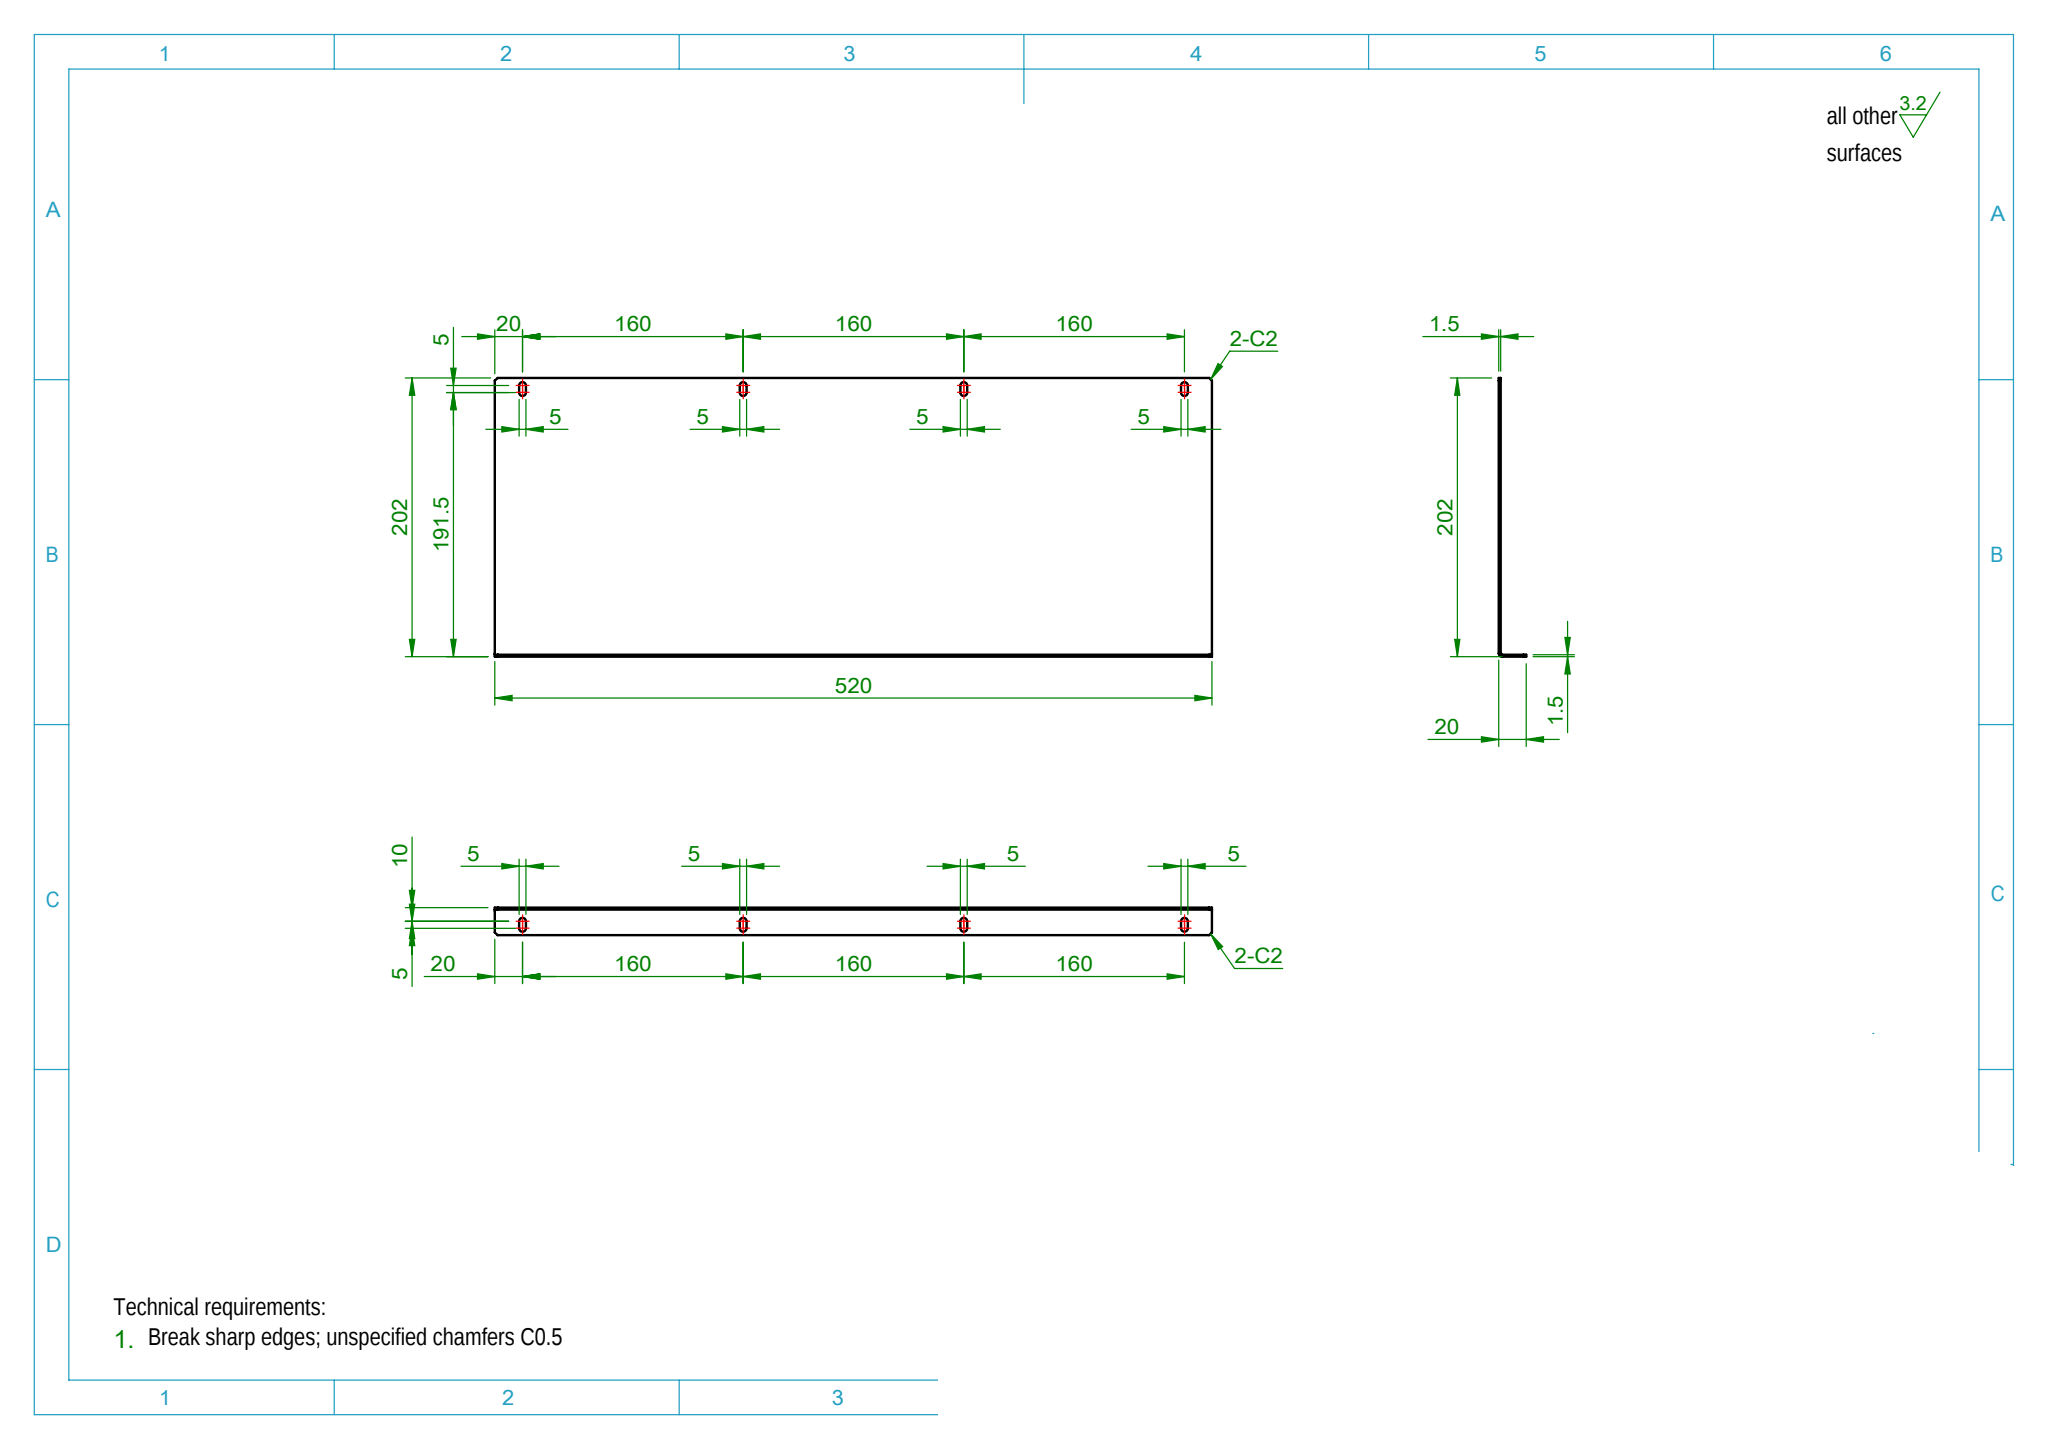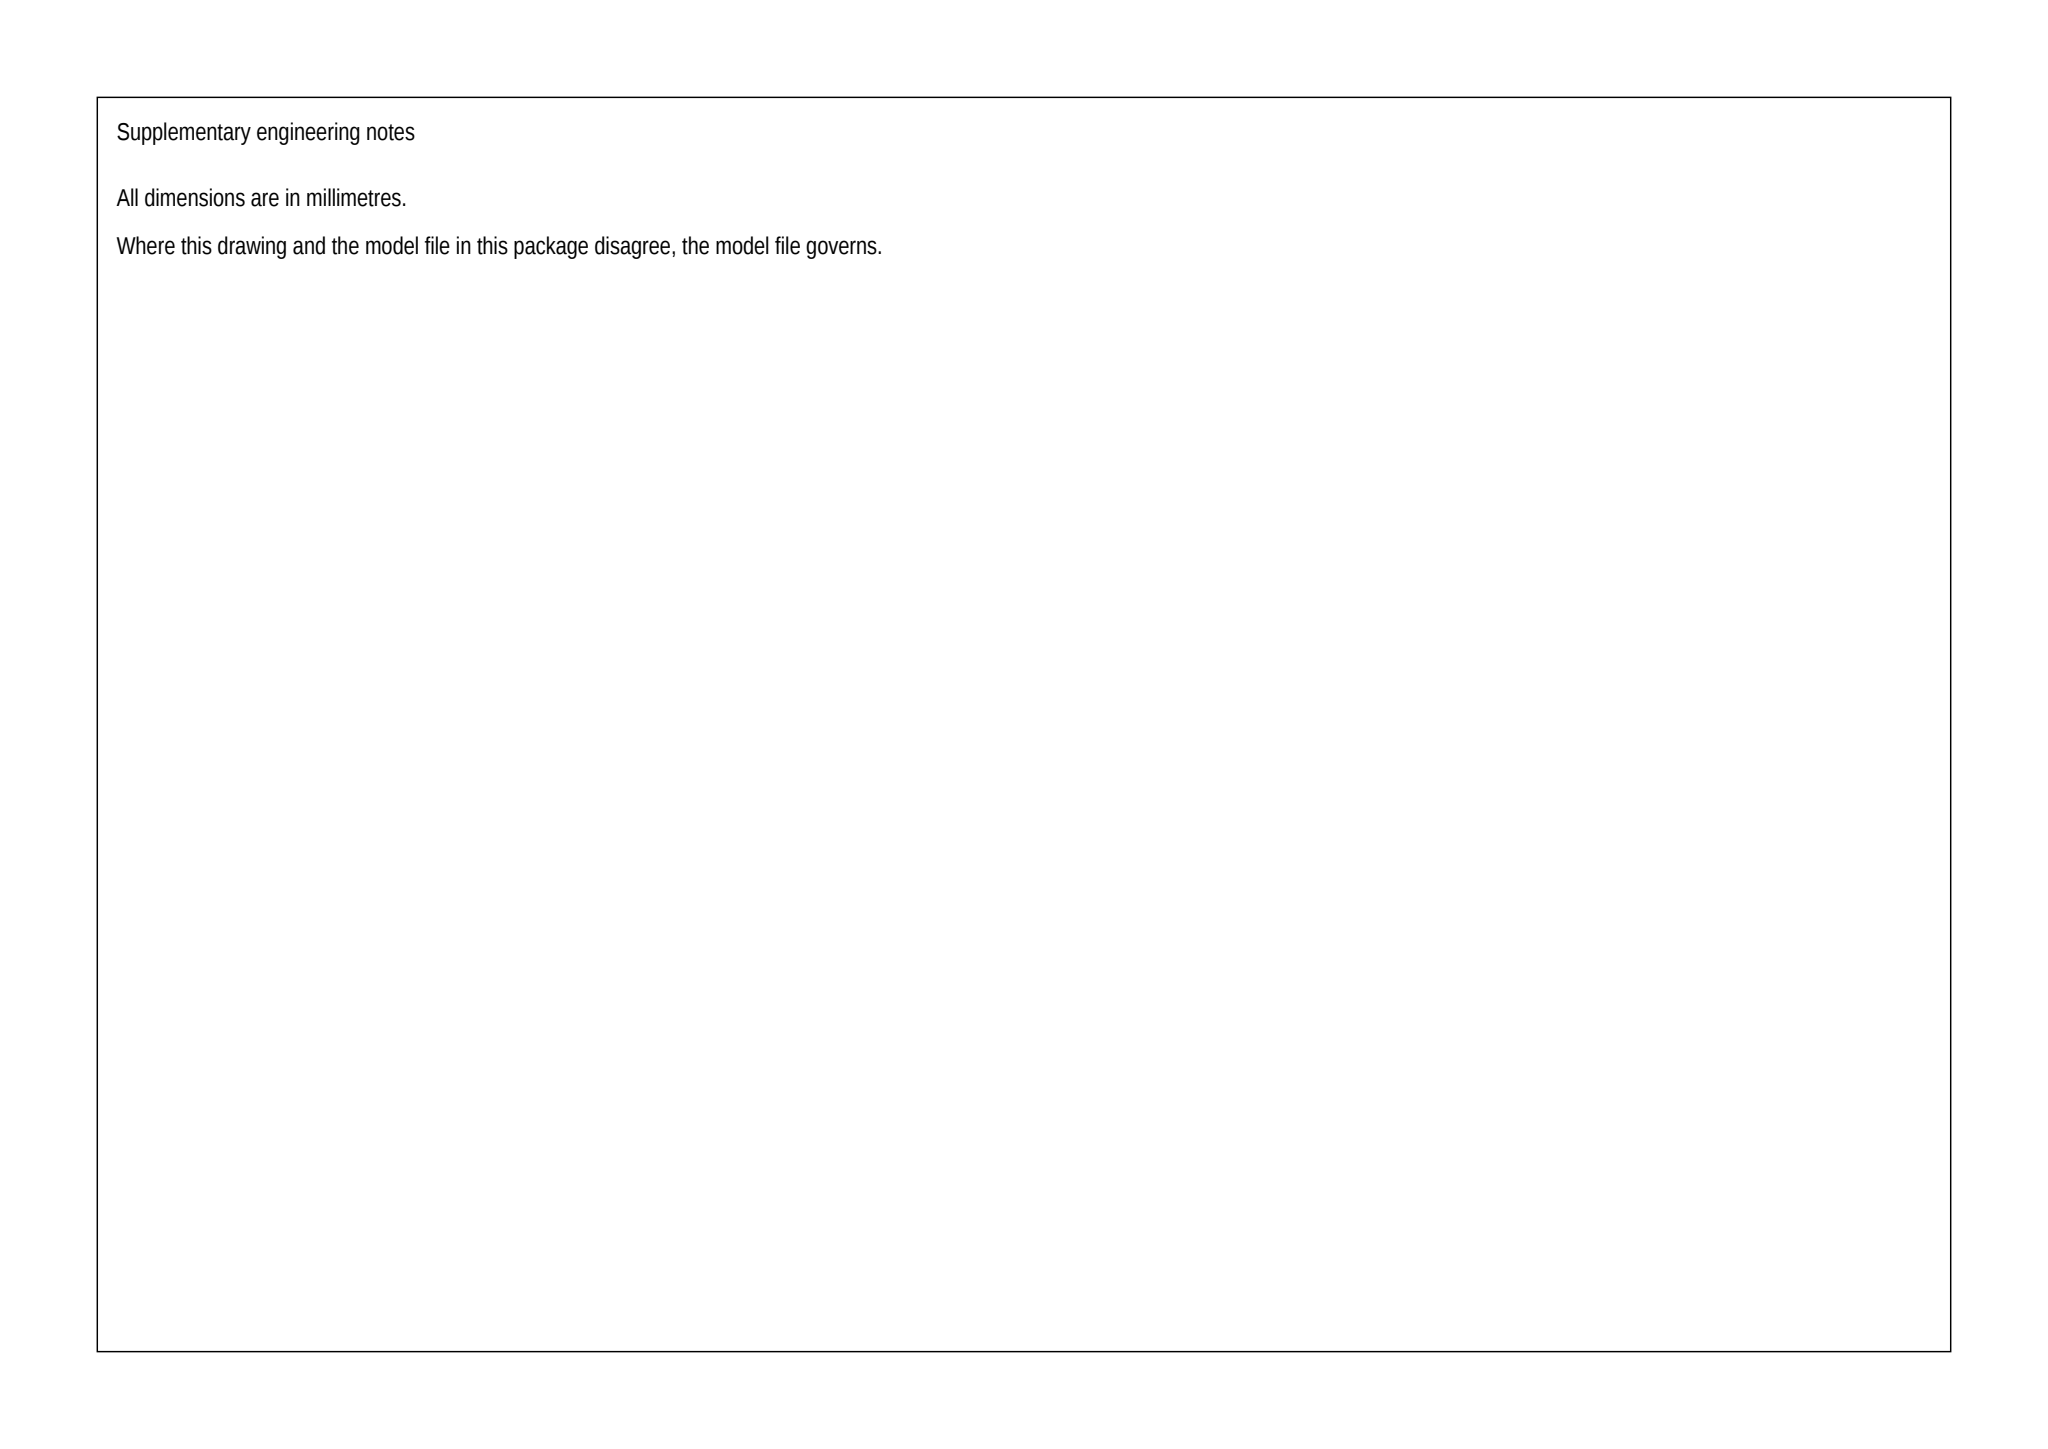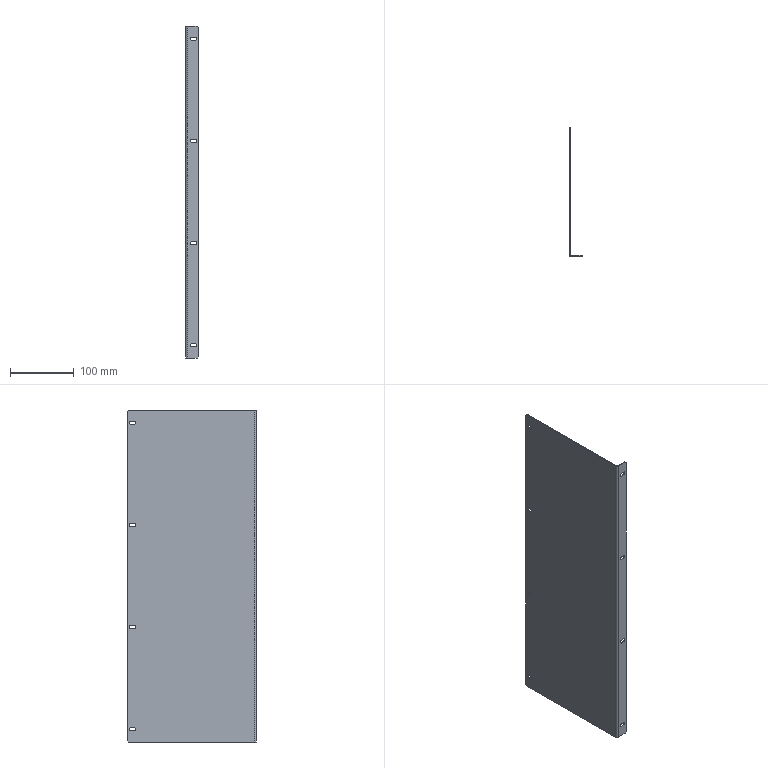Part | SolidWorks | mm | 1 solid | 54 faces | box 20 x 202 x 520 mm | volume 170857 mm3 | plane 32 | cylinder 22 | commonest cylinder face diameters 5 x21 2 x1